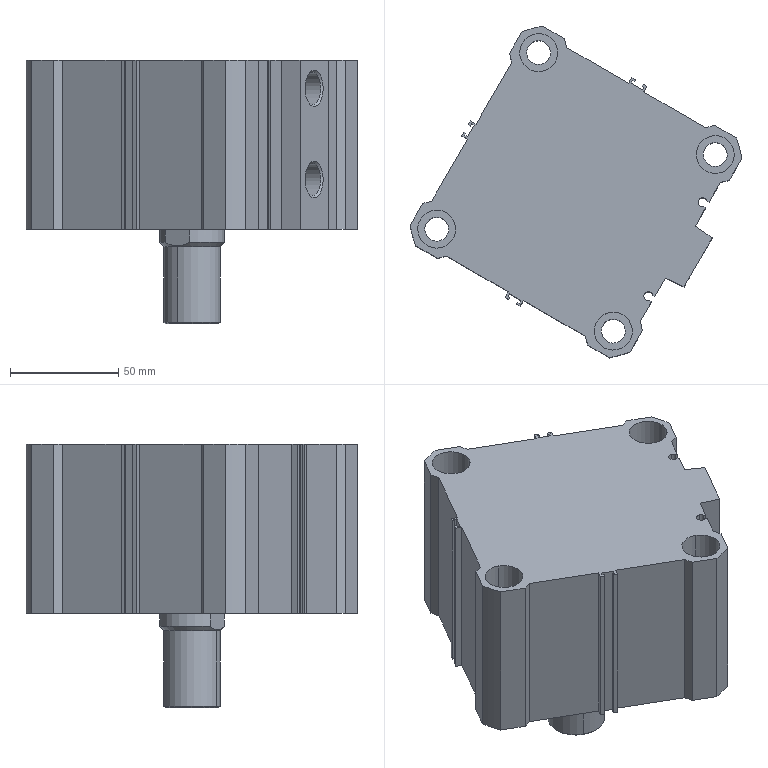Component | SolidWorks | SpindleFixtureAssemblyLeft-1_A_CDQ2B100-15DM(0)-1 | 2 solids | 137 faces | volume 960681 mm3 | plane 83 | cylinder 44 | cone 8 | spline 2 | commonest cylinder face diameters 17.5 x16 11 x8 4.2 x6 14.95 x4 156 x4 30.4 x2 26 x2 30 x2